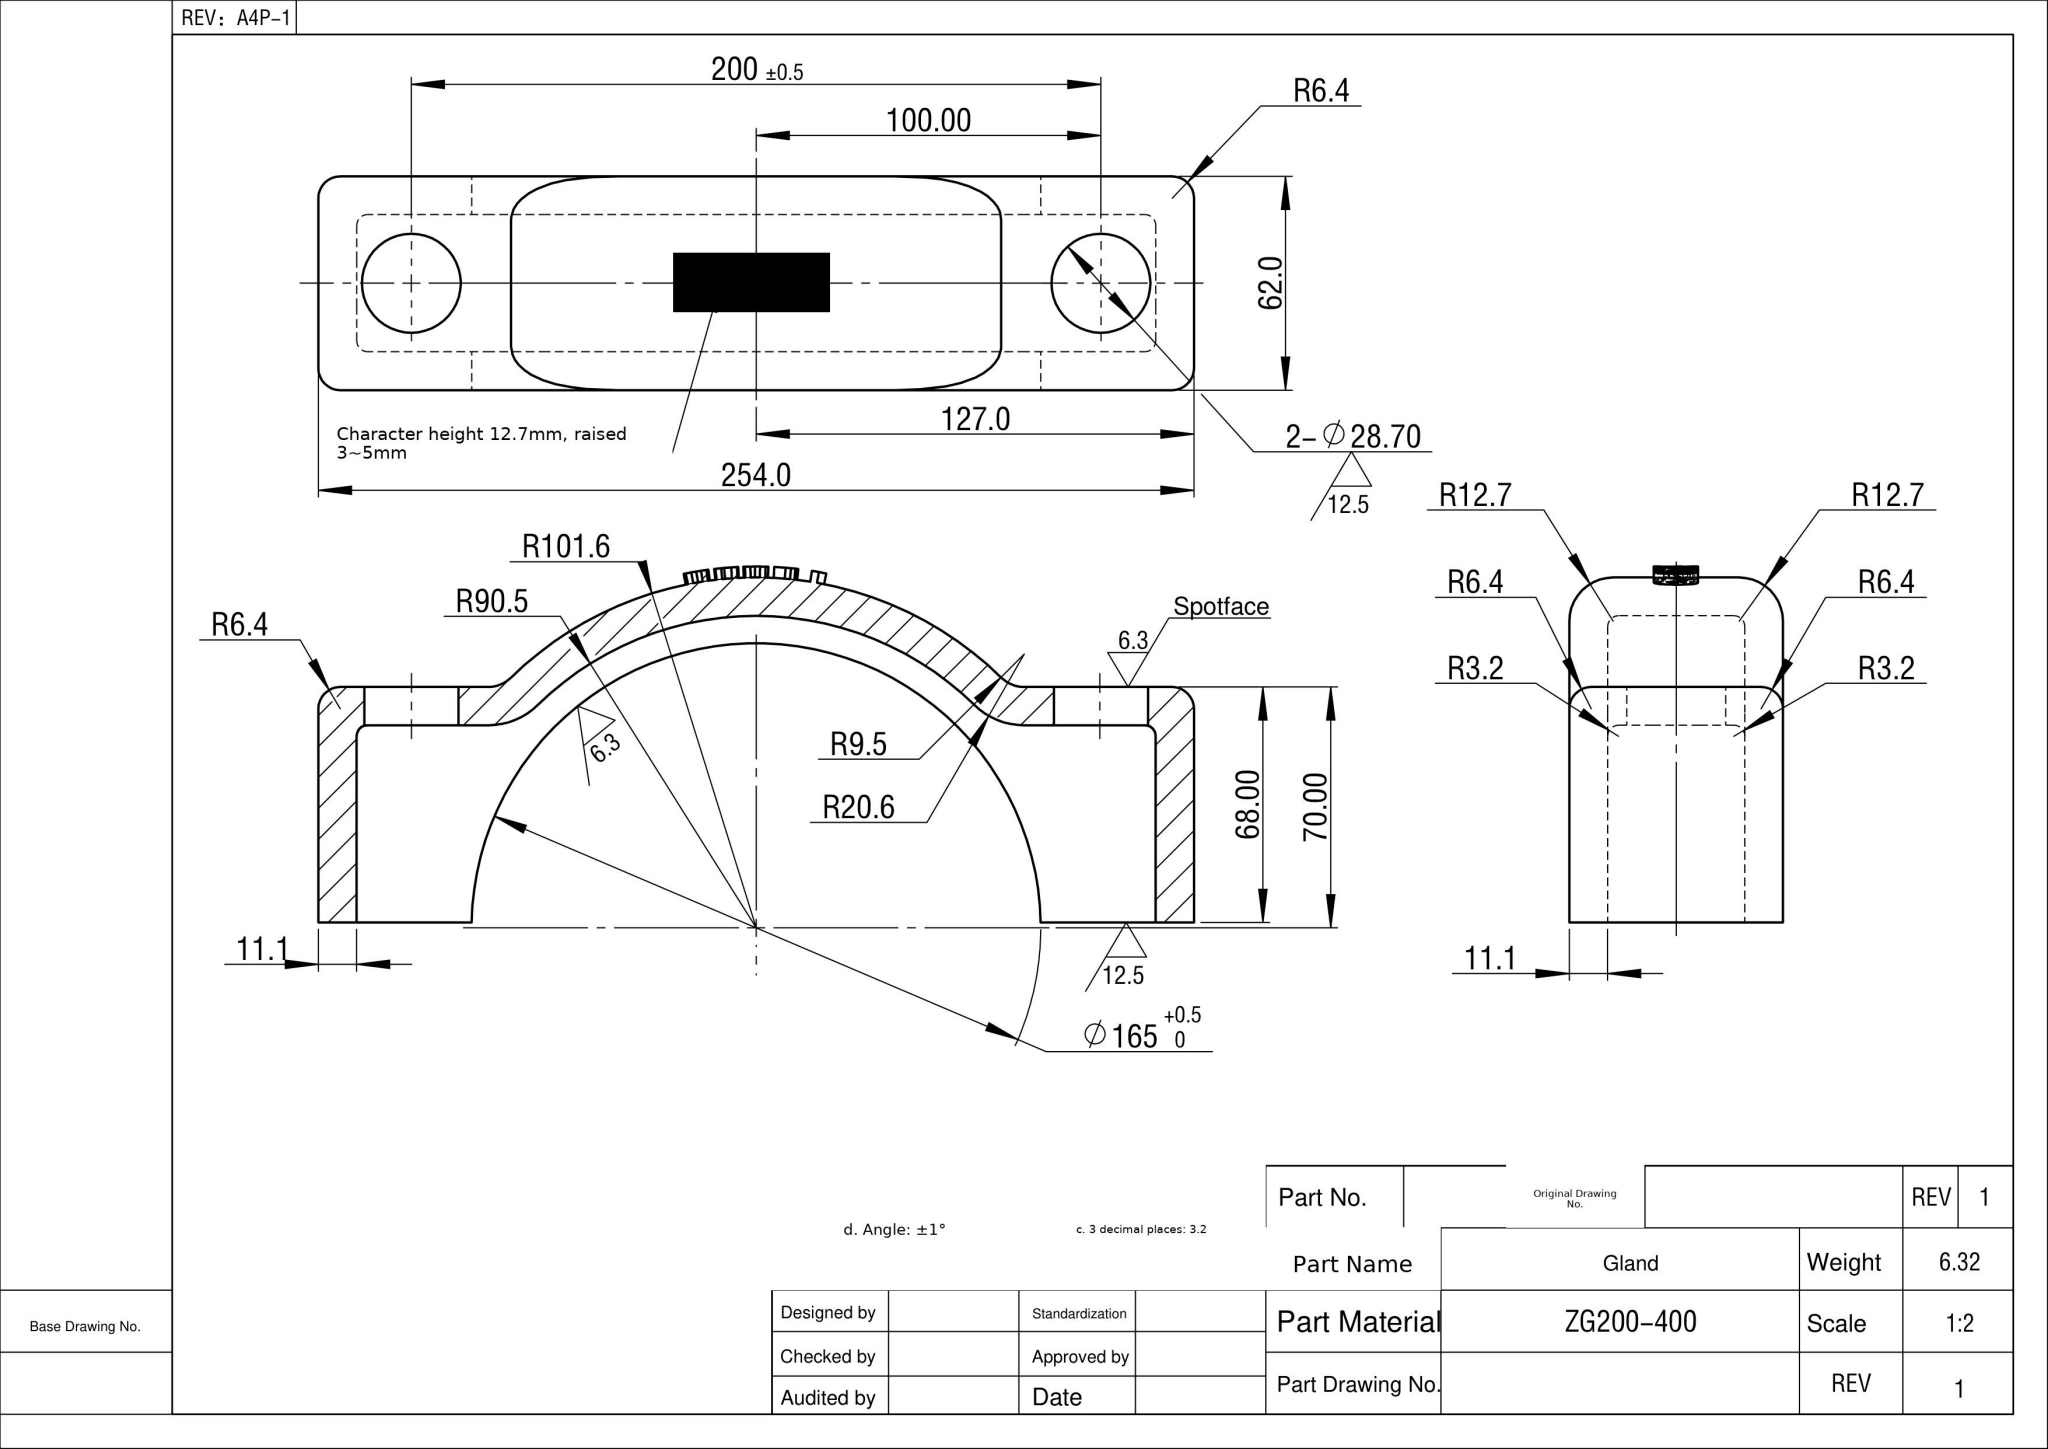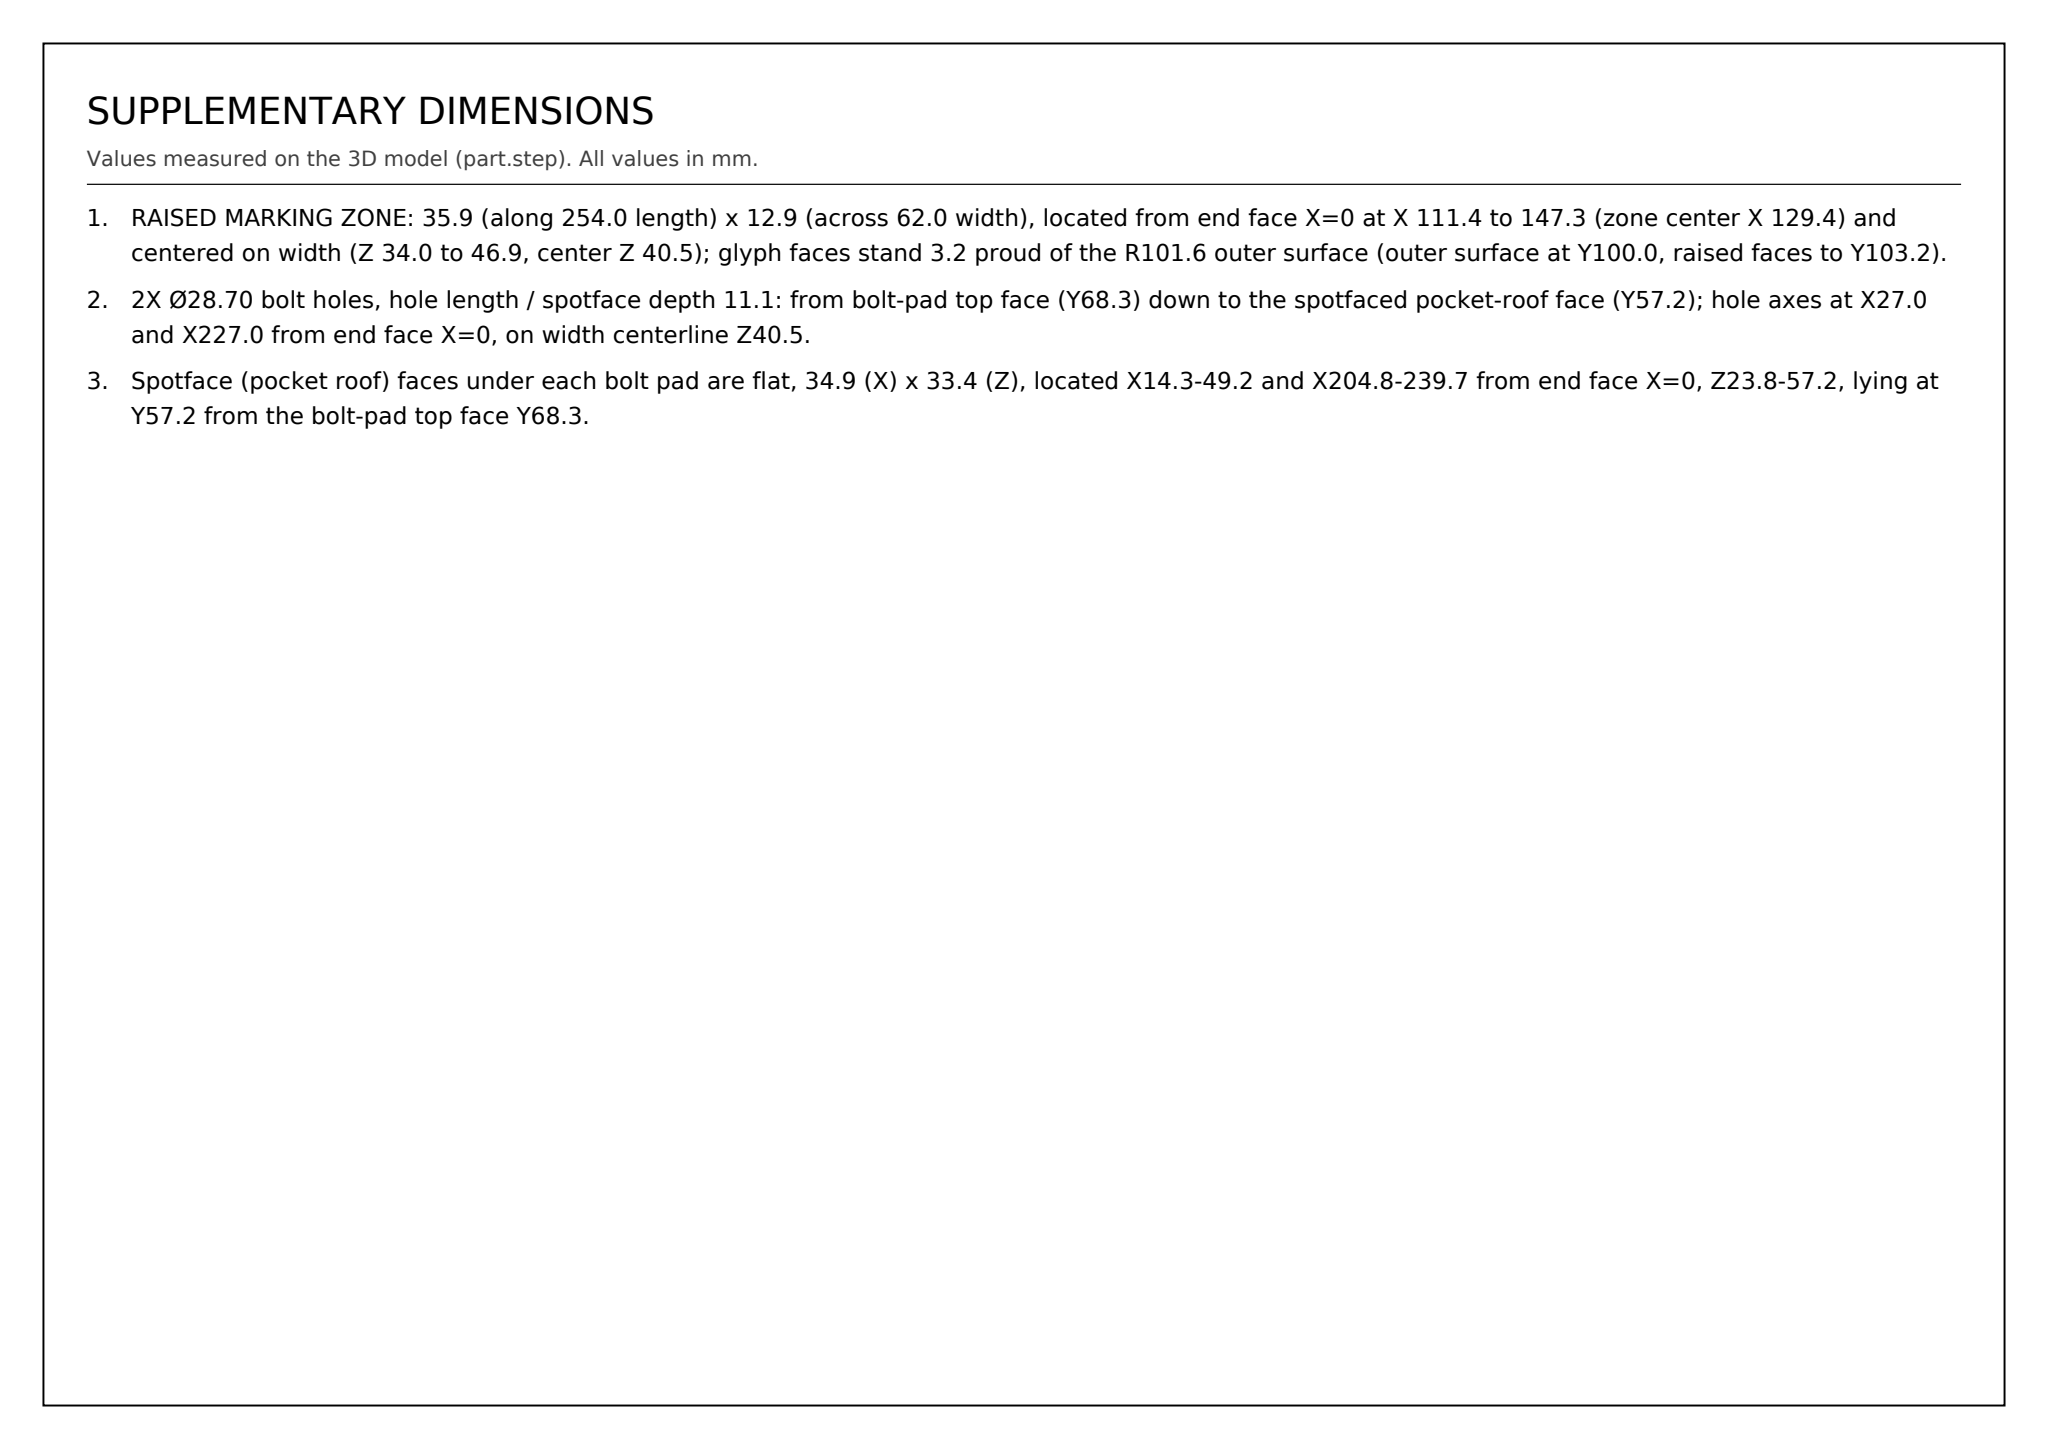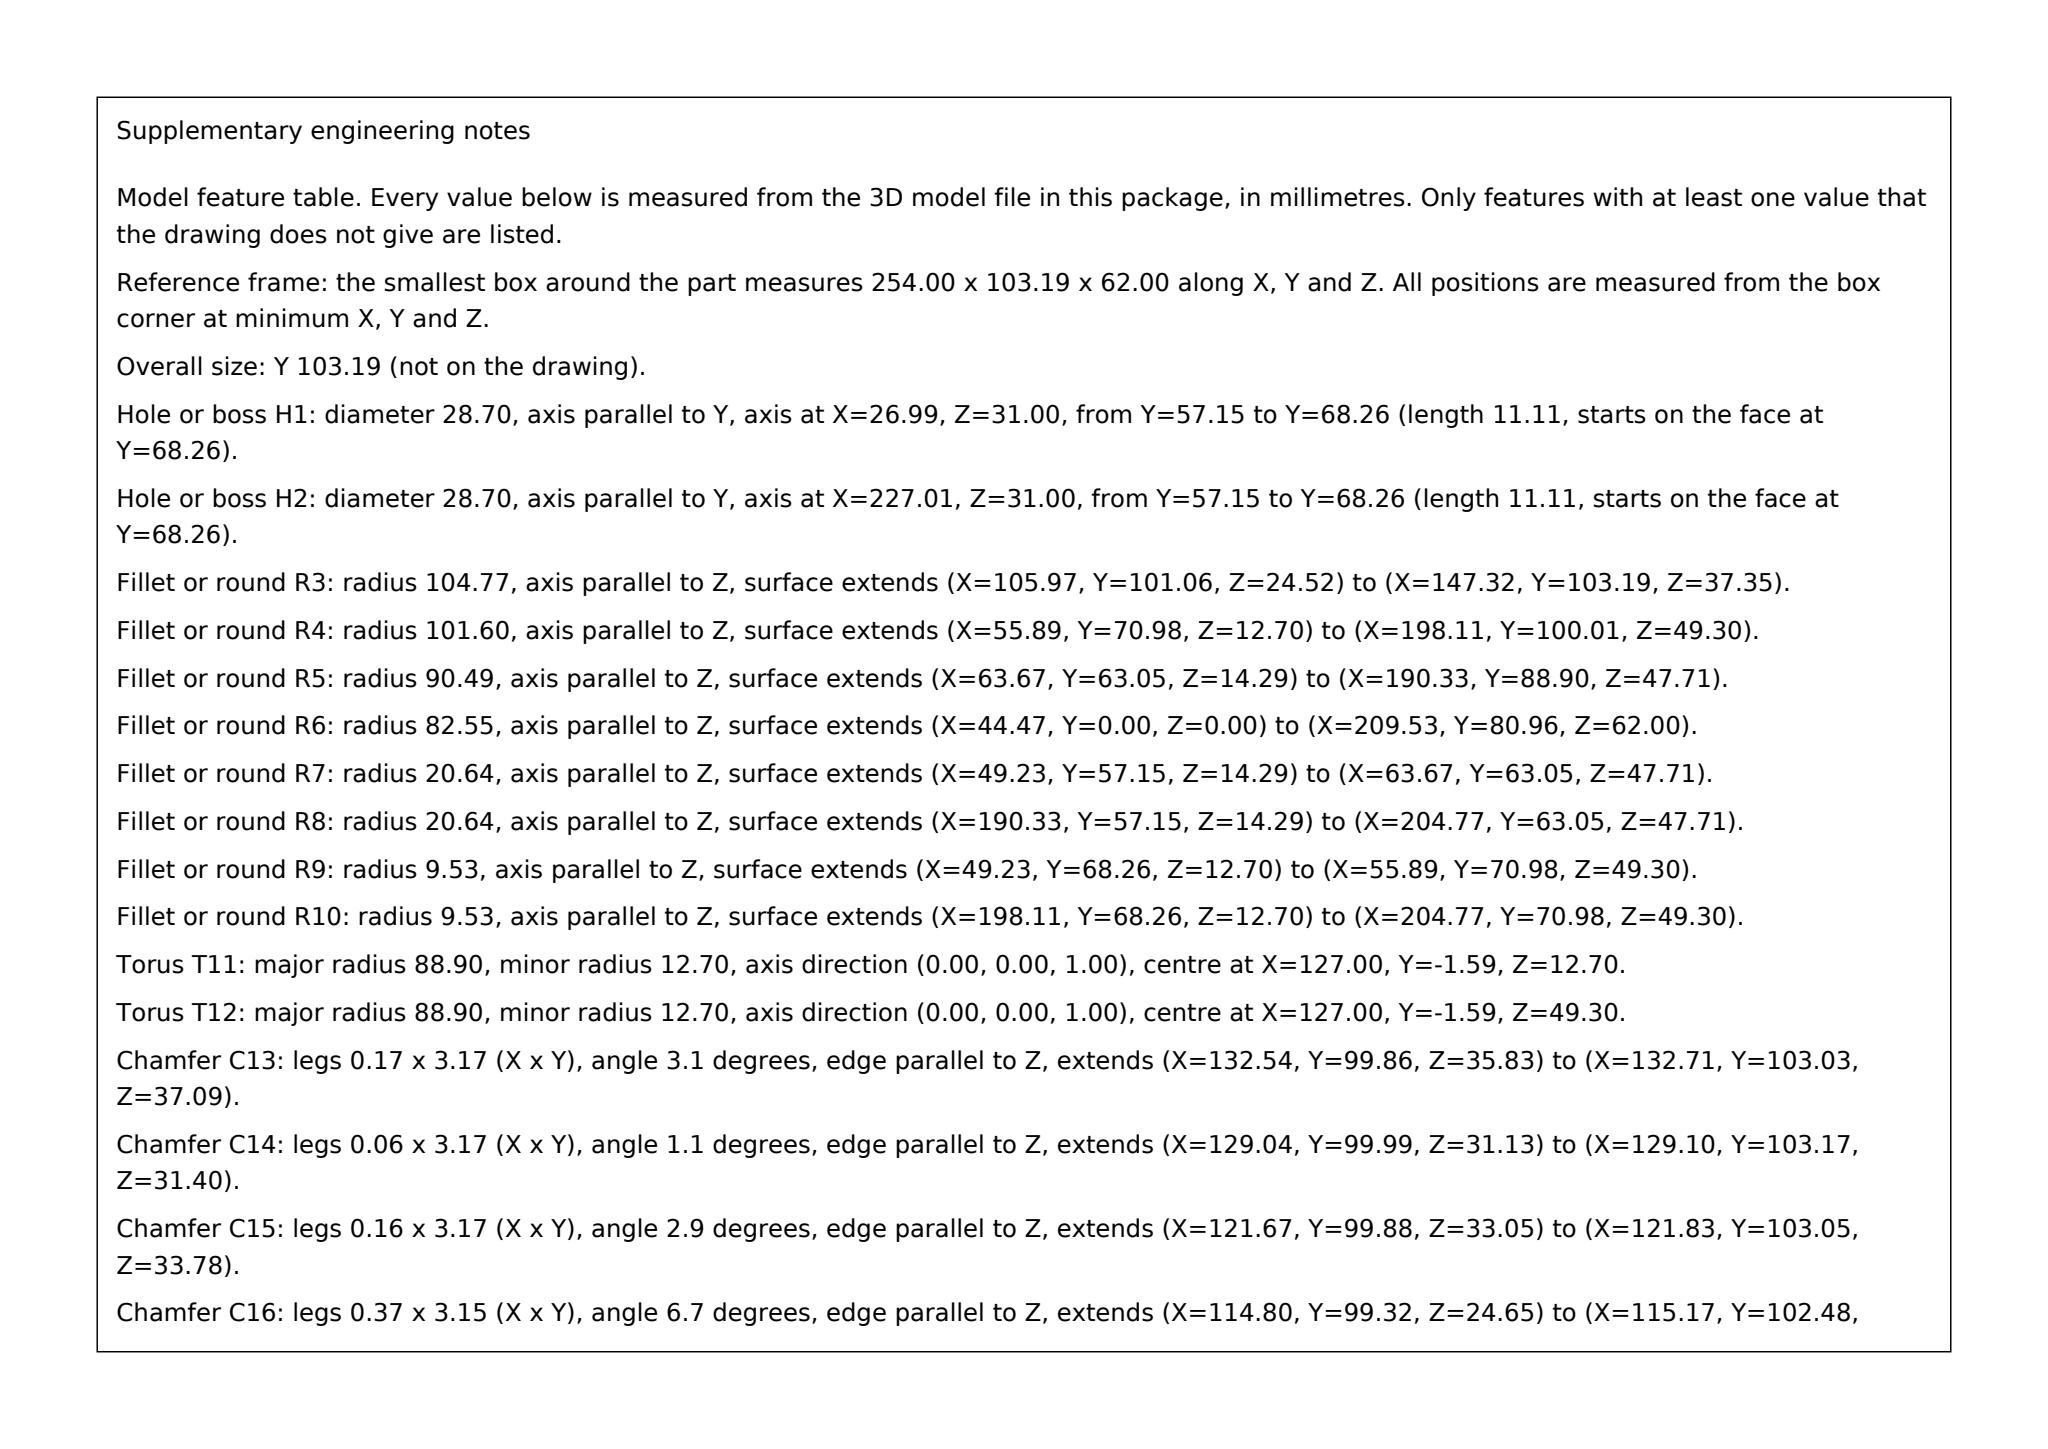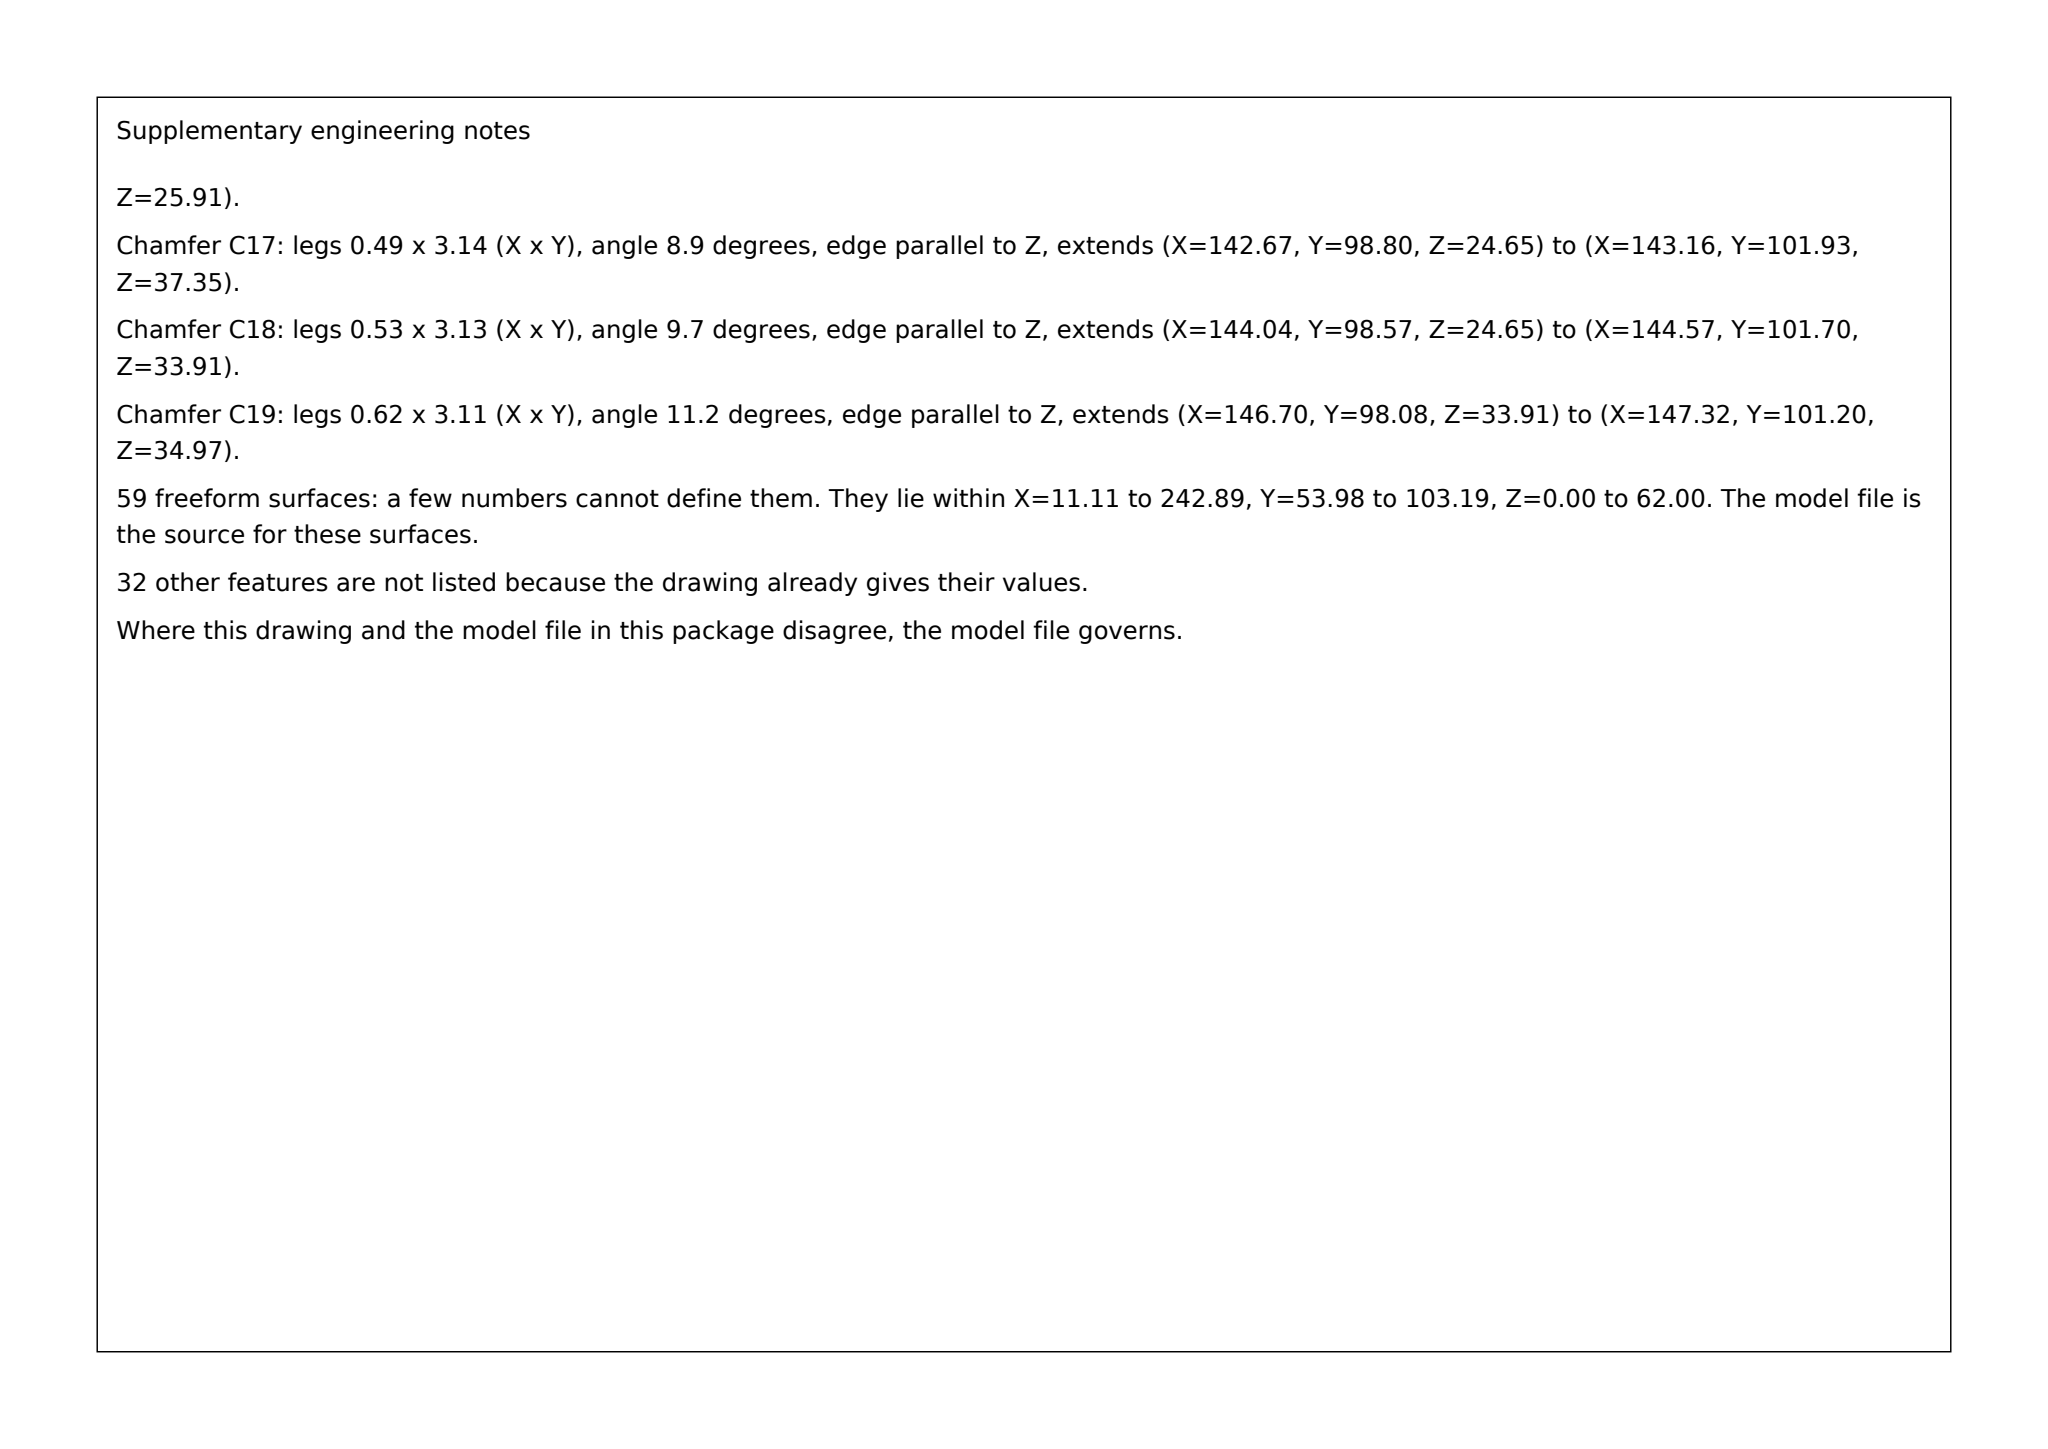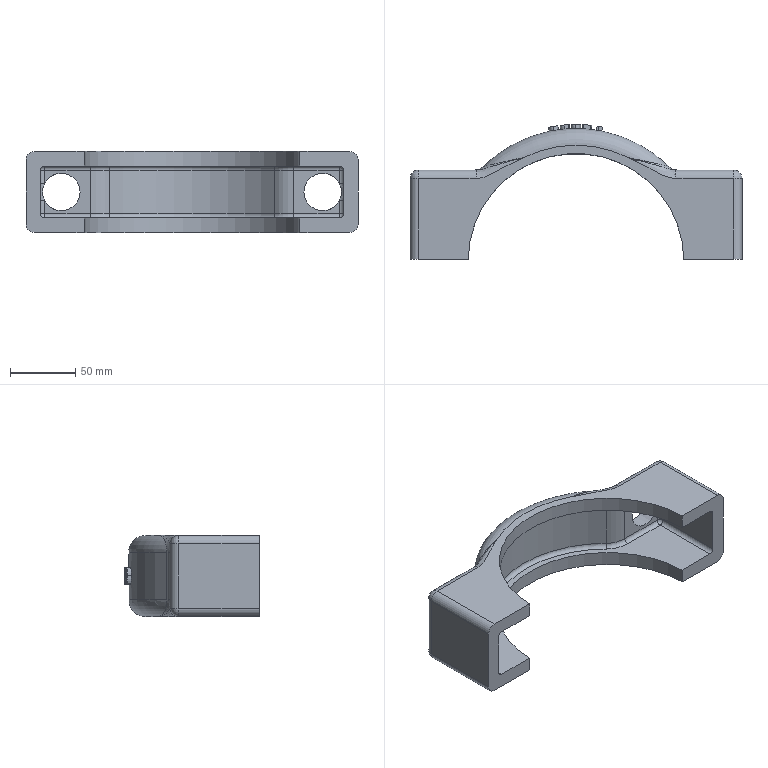Part | SolidWorks | mm | 1 solid | 150 faces | box 254 x 103.19 x 62 mm | volume 367497 mm3 | spline 59 | cylinder 41 | plane 34 | torus 8 | sphere 8 | commonest cylinder face diameters 6.35 x12 12.7 x10 209.55 x5 28.702 x4 203.2 x3 165.1 x2 19.05 x2 41.275 x2
Drawing notes:
RAISED MARKING ZONE: 35.9 (along 254.0 length) x 12.9 (across 62.0 width), located from end face X=0 at X 111.4 to 147.3 (zone center X 129.4) and centered on width (Z 34.0 to 46.9, center Z 40.5); glyph faces stand 3.2 proud of the R101.6 outer surface (outer surface at Y100.0, raised faces to Y103.2). | from the solid: axis_planes z=34.2..46.9 groups with x extents 111.4-147.3 and y 98.1-103.2 (raised glyph faces) plus inclined_planes bbox_from x111.4-146.7, y98.1-100.0, z34.2-46.9; convex arc dia 203.2 (R101.6) axis z at [127.0,-1.6]
2X Ø28.70 bolt holes, hole length / spotface depth 11.1: from bolt-pad top face (Y68.3) down to the spotfaced pocket-roof face (Y57.2); hole axes at X27.0 and X227.0 from end face X=0, on width centerline Z40.5. | from the solid: cylinders: hole/bore dia 28.7, axis y, at (227.0,40.5) and (27.0,40.5), from y57.2 to y68.3; axis_planes y=68.3 (pad top, x6.4-50.6 / 203.4-247.7) and y=57.2 (spotface, x14.3-49.2 / 204.8-239.7)
Spotface (pocket roof) faces under each bolt pad are flat, 34.9 (X) x 33.4 (Z), located X14.3-49.2 and X204.8-239.7 from end face X=0, Z23.8-57.2, lying at Y57.2 from the bolt-pad top face Y68.3. | from the solid: axis_planes y=57.2 extent x[14.3,49.2] z[23.8,57.2] area 536 and x[204.8,239.7] z[23.8,57.2] area 536